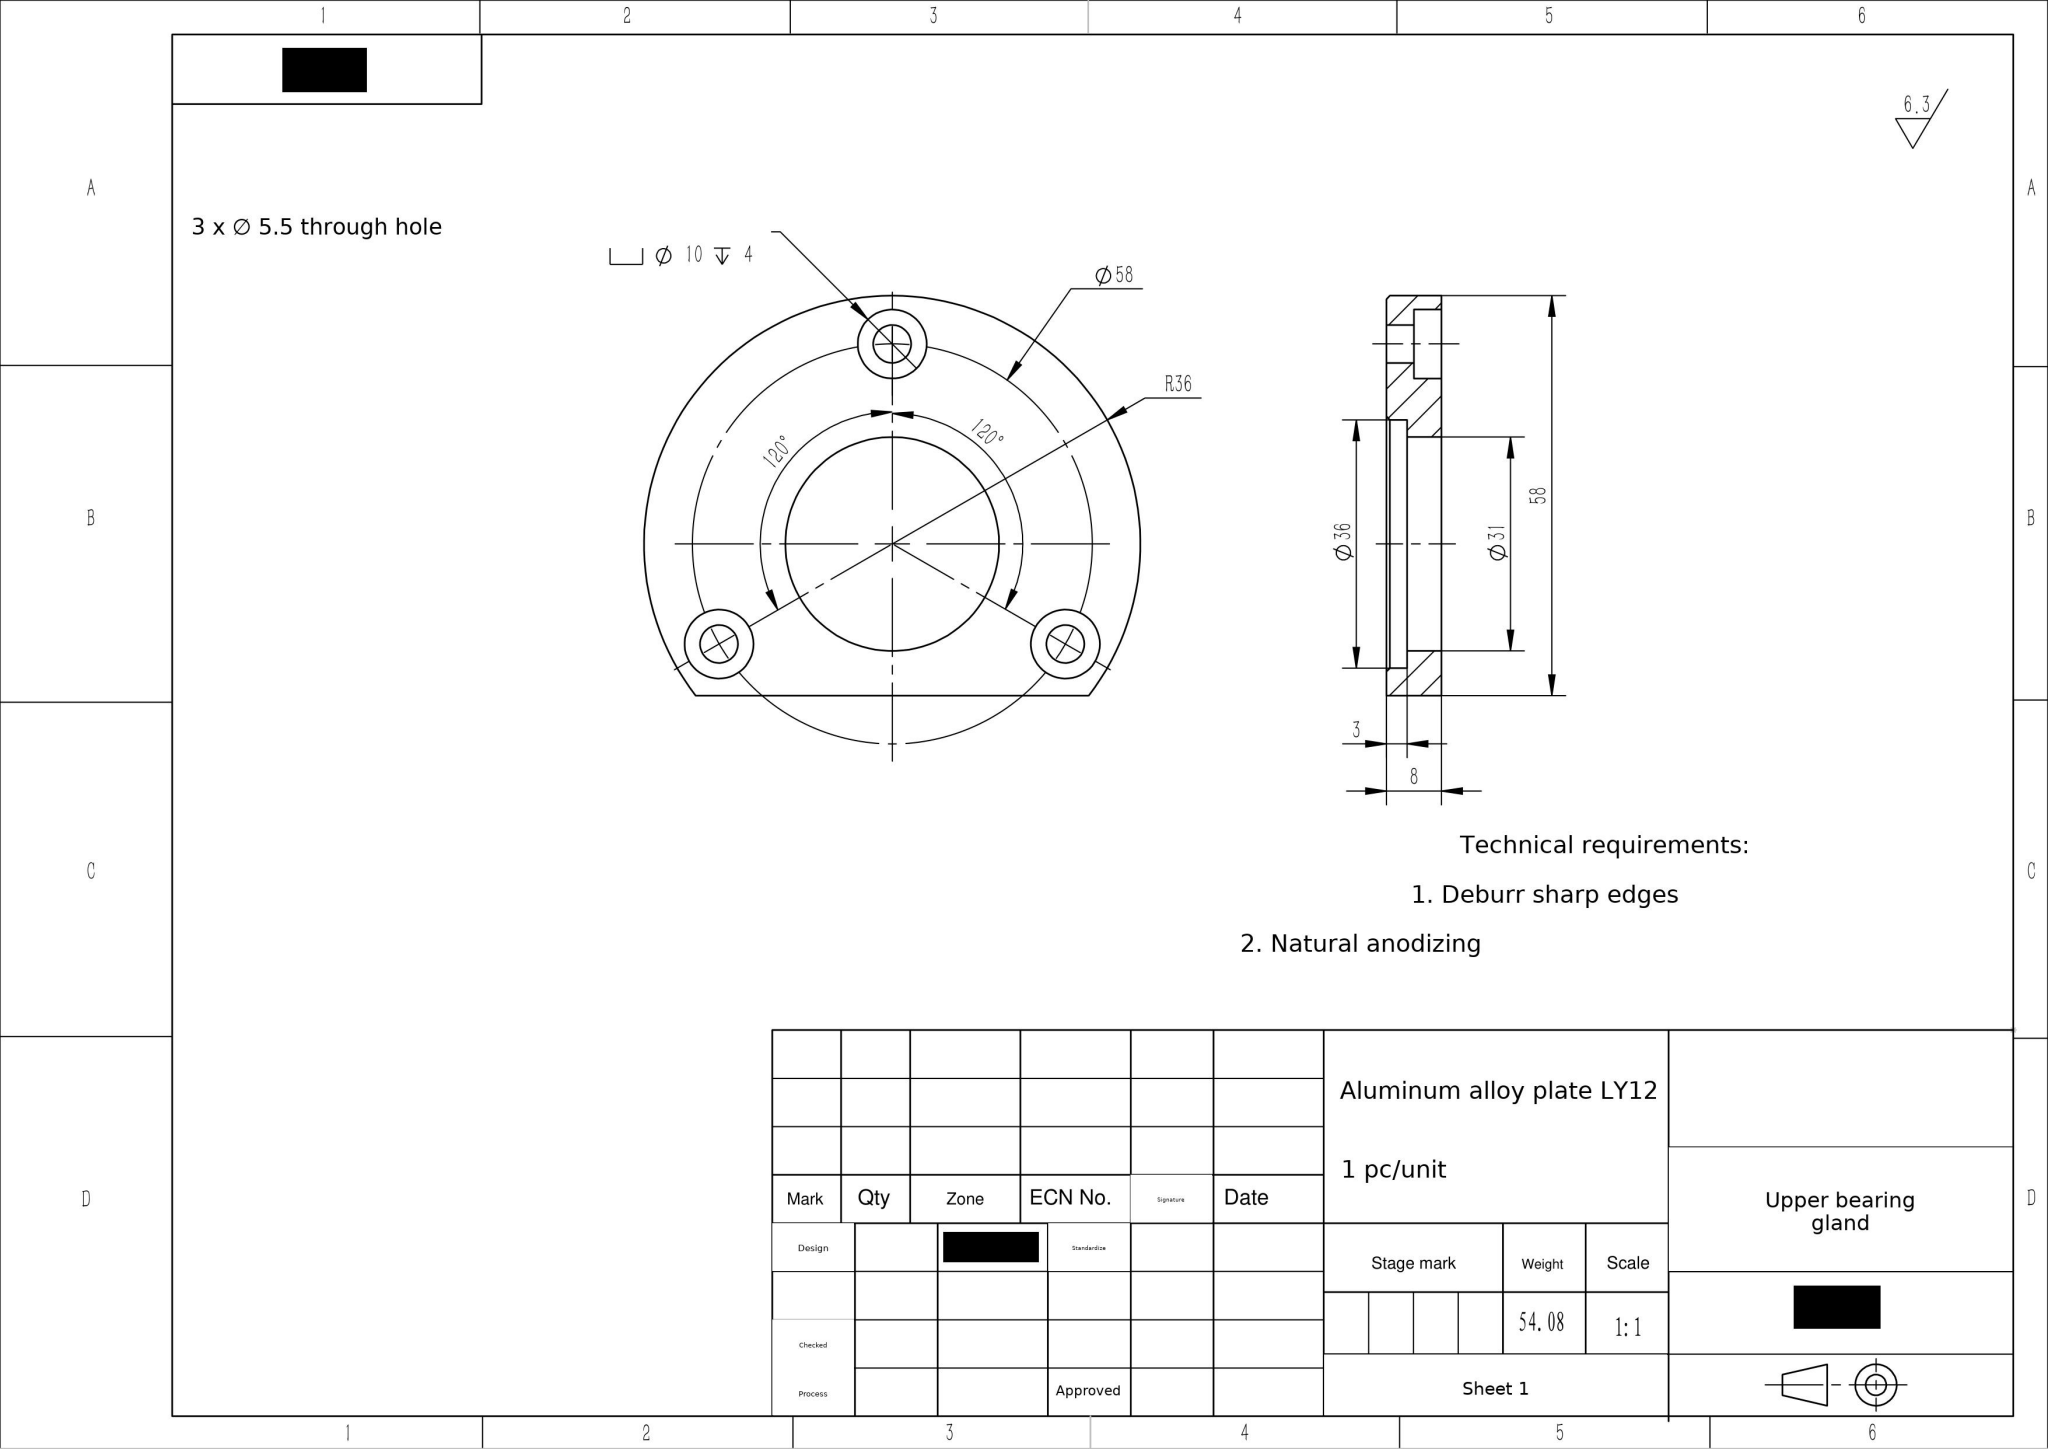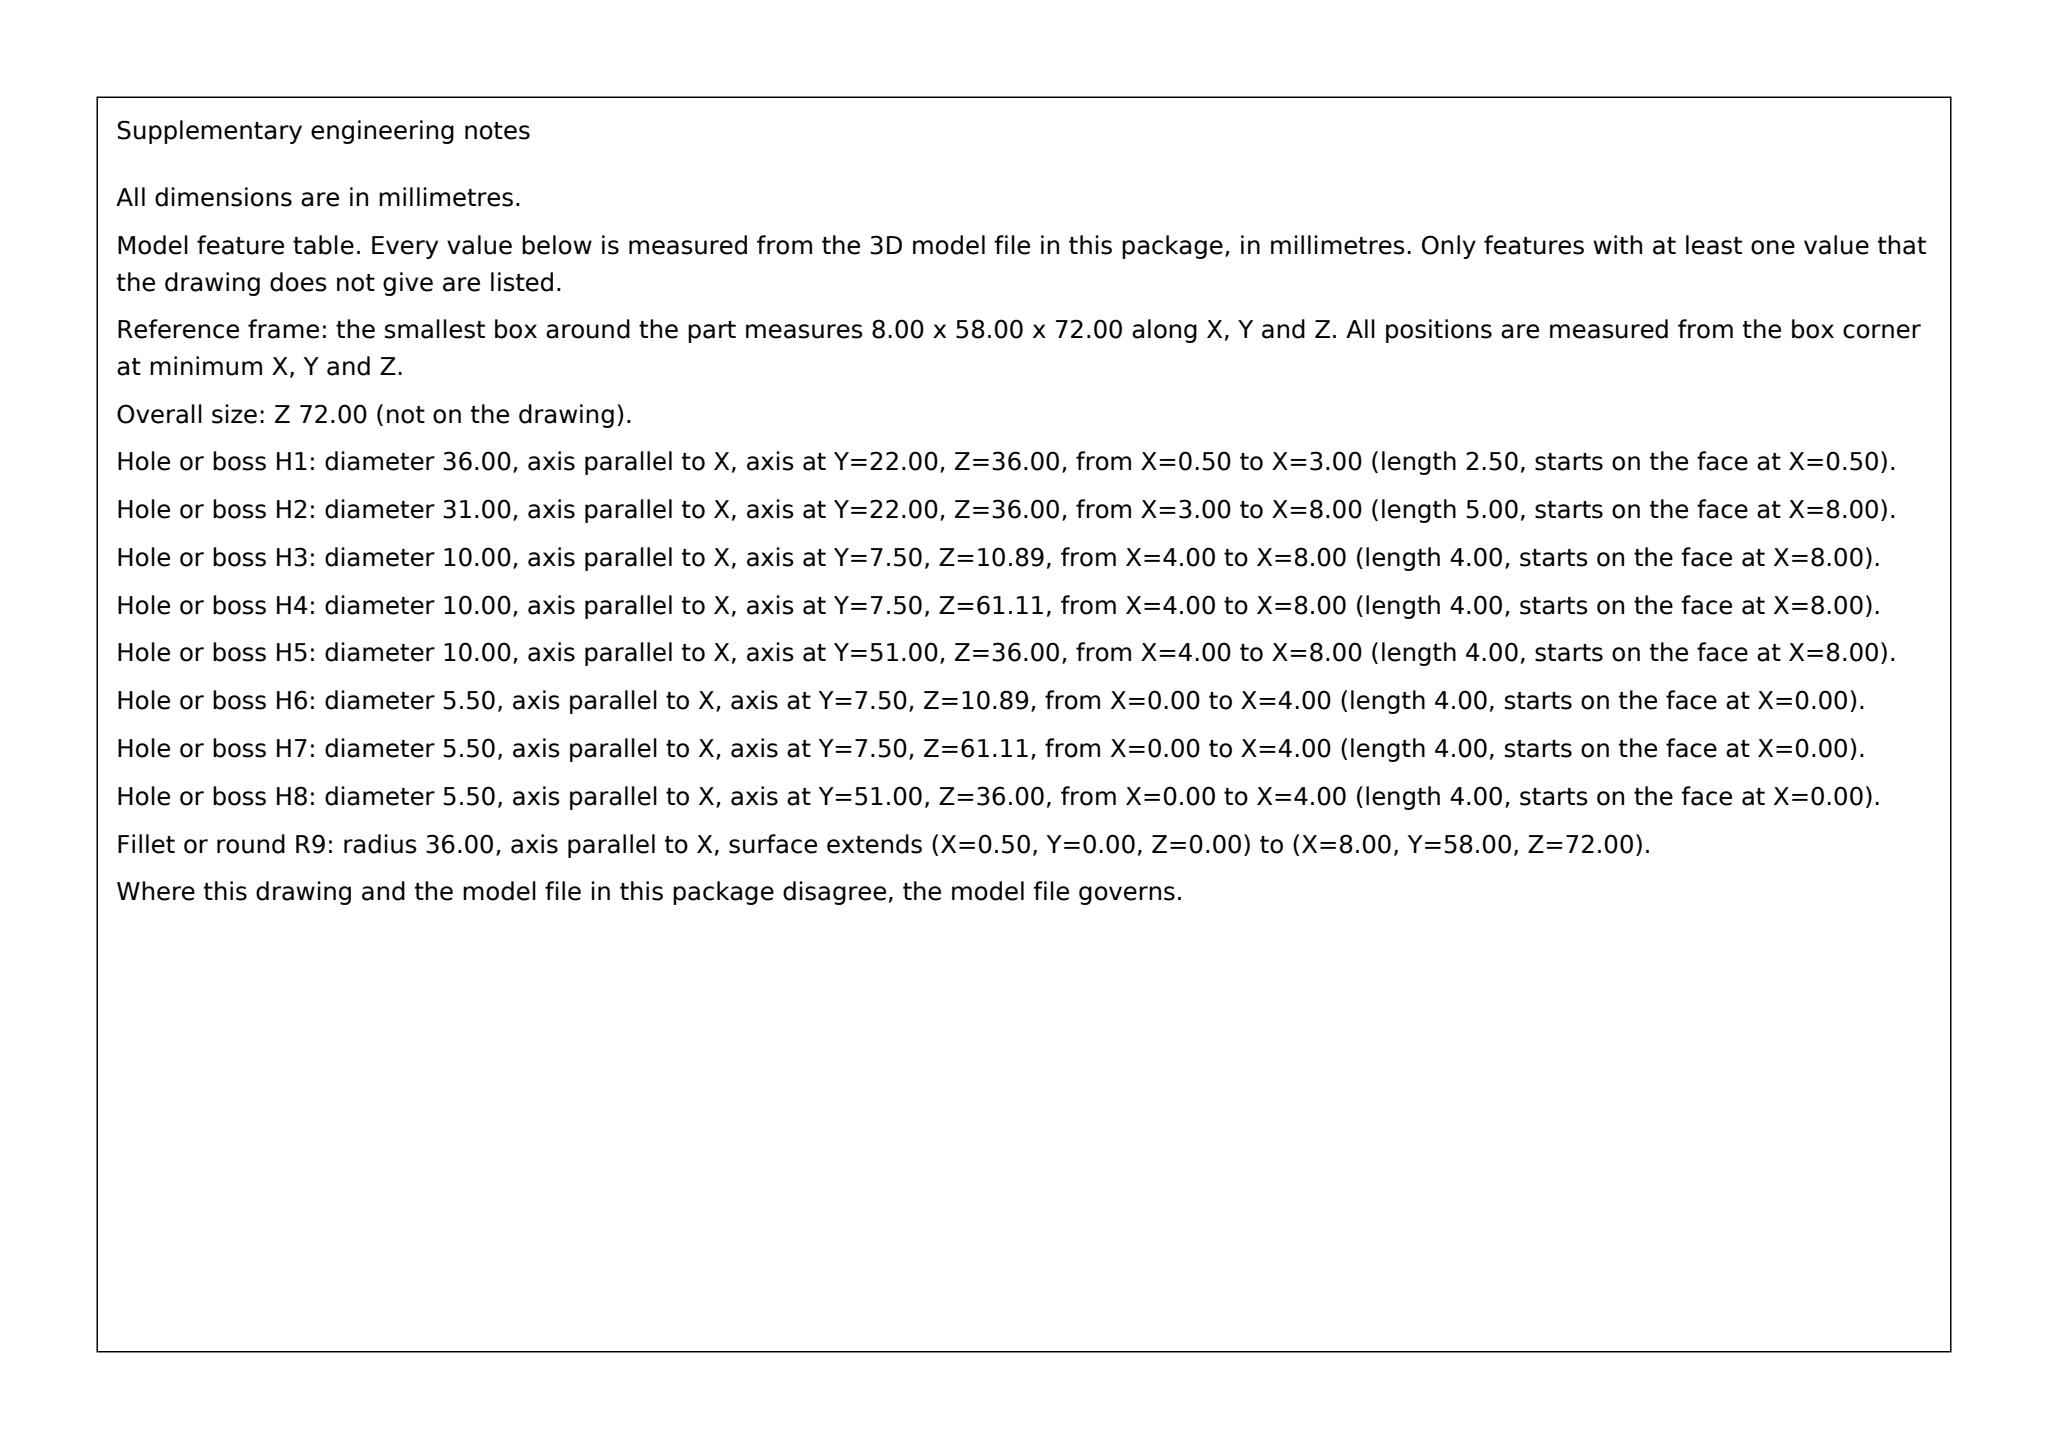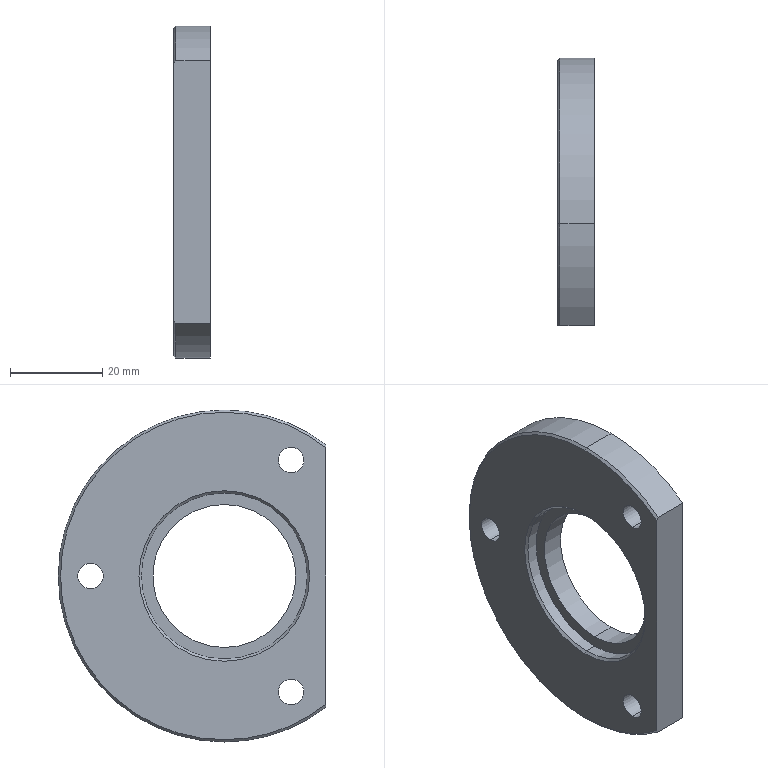Part | SolidWorks | mm | material Aluminum alloy plate LY12 | 1 solid | 31 faces | box 8 x 58 x 72 mm | volume 20029 mm3 | cylinder 19 | plane 7 | cone 5 | commonest cylinder face diameters 10 x6 5.5 x6 72 x3 31 x2 36 x2
build123d program:
from build123d import *

# Parameters (mm, degrees)
M5_HEX_SOCKET_HEAD_CAP_SCREW_CBORE1_D           = 5.5
M5_HEX_SOCKET_HEAD_CAP_SCREW_CBORE1_CBORE_D     = 10
M5_HEX_SOCKET_HEAD_CAP_SCREW_CBORE1_CBORE_DEPTH = 4
CIRPATTERN1_COUNT                               = 3
CHAMFER1_SIZE                                   = 0.5
SKETCH4_W                                       = 100
SKETCH4_H                                       = 23.071
CUT_EXTRUDE1_DEPTH                              = 52.536


with BuildPart() as part:
    # Sketch1 → Revolve1 (revolve)
    with BuildSketch(Plane.XY, mode=Mode.PRIVATE) as revolve1_sk:
        Polygon((0, 36), (0, 18), (3, 18), (3, 15.5), (8, 15.5), (8, 36), align=None)
    revolve(revolve1_sk.sketch.rotate(Axis((-16.971, 0, 0), (1, 0, 0)), 90), axis=Axis((-16.971, 0, 0), (1, 0, 0)))

    # M5 Hex Socket Head Cap Screw CBORE1 (through all)
    with Locations(Plane(origin=(8, 0, 0), x_dir=(0, 0, -1), z_dir=(1, 0, 0))):
        with Locations((0, 29)):
            m5_hex_socket_head_cap_screw_cbore1 = CounterBoreHole(M5_HEX_SOCKET_HEAD_CAP_SCREW_CBORE1_D / 2, M5_HEX_SOCKET_HEAD_CAP_SCREW_CBORE1_CBORE_D / 2, M5_HEX_SOCKET_HEAD_CAP_SCREW_CBORE1_CBORE_DEPTH)

    # CirPattern1: M5 Hex Socket Head Cap Screw CBORE1 ×3 about axis
    cirpattern1_axis = Axis((0, 0, 0), (1, 0, 0))
    for i in range(1, CIRPATTERN1_COUNT):
        add(m5_hex_socket_head_cap_screw_cbore1.rotate(cirpattern1_axis, i * 360 / CIRPATTERN1_COUNT), mode=Mode.SUBTRACT)

    # Chamfer1
    chamfer1_edges = [part.edges().sort_by_distance(p)[0] for p in [
        (0, 0, -18),
        (0, 0, -36),
    ]]
    chamfer(chamfer1_edges, length=CHAMFER1_SIZE)

    # Sketch4 → Cut-Extrude1 (cut, through all)
    with BuildSketch(Plane(origin=(8, 0, 0), x_dir=(0, 0, -1), z_dir=(1, 0, 0))):
        with Locations((0, -33.536)):
            Rectangle(SKETCH4_W, SKETCH4_H)
    extrude(amount=-CUT_EXTRUDE1_DEPTH, mode=Mode.SUBTRACT)


solid = part.part